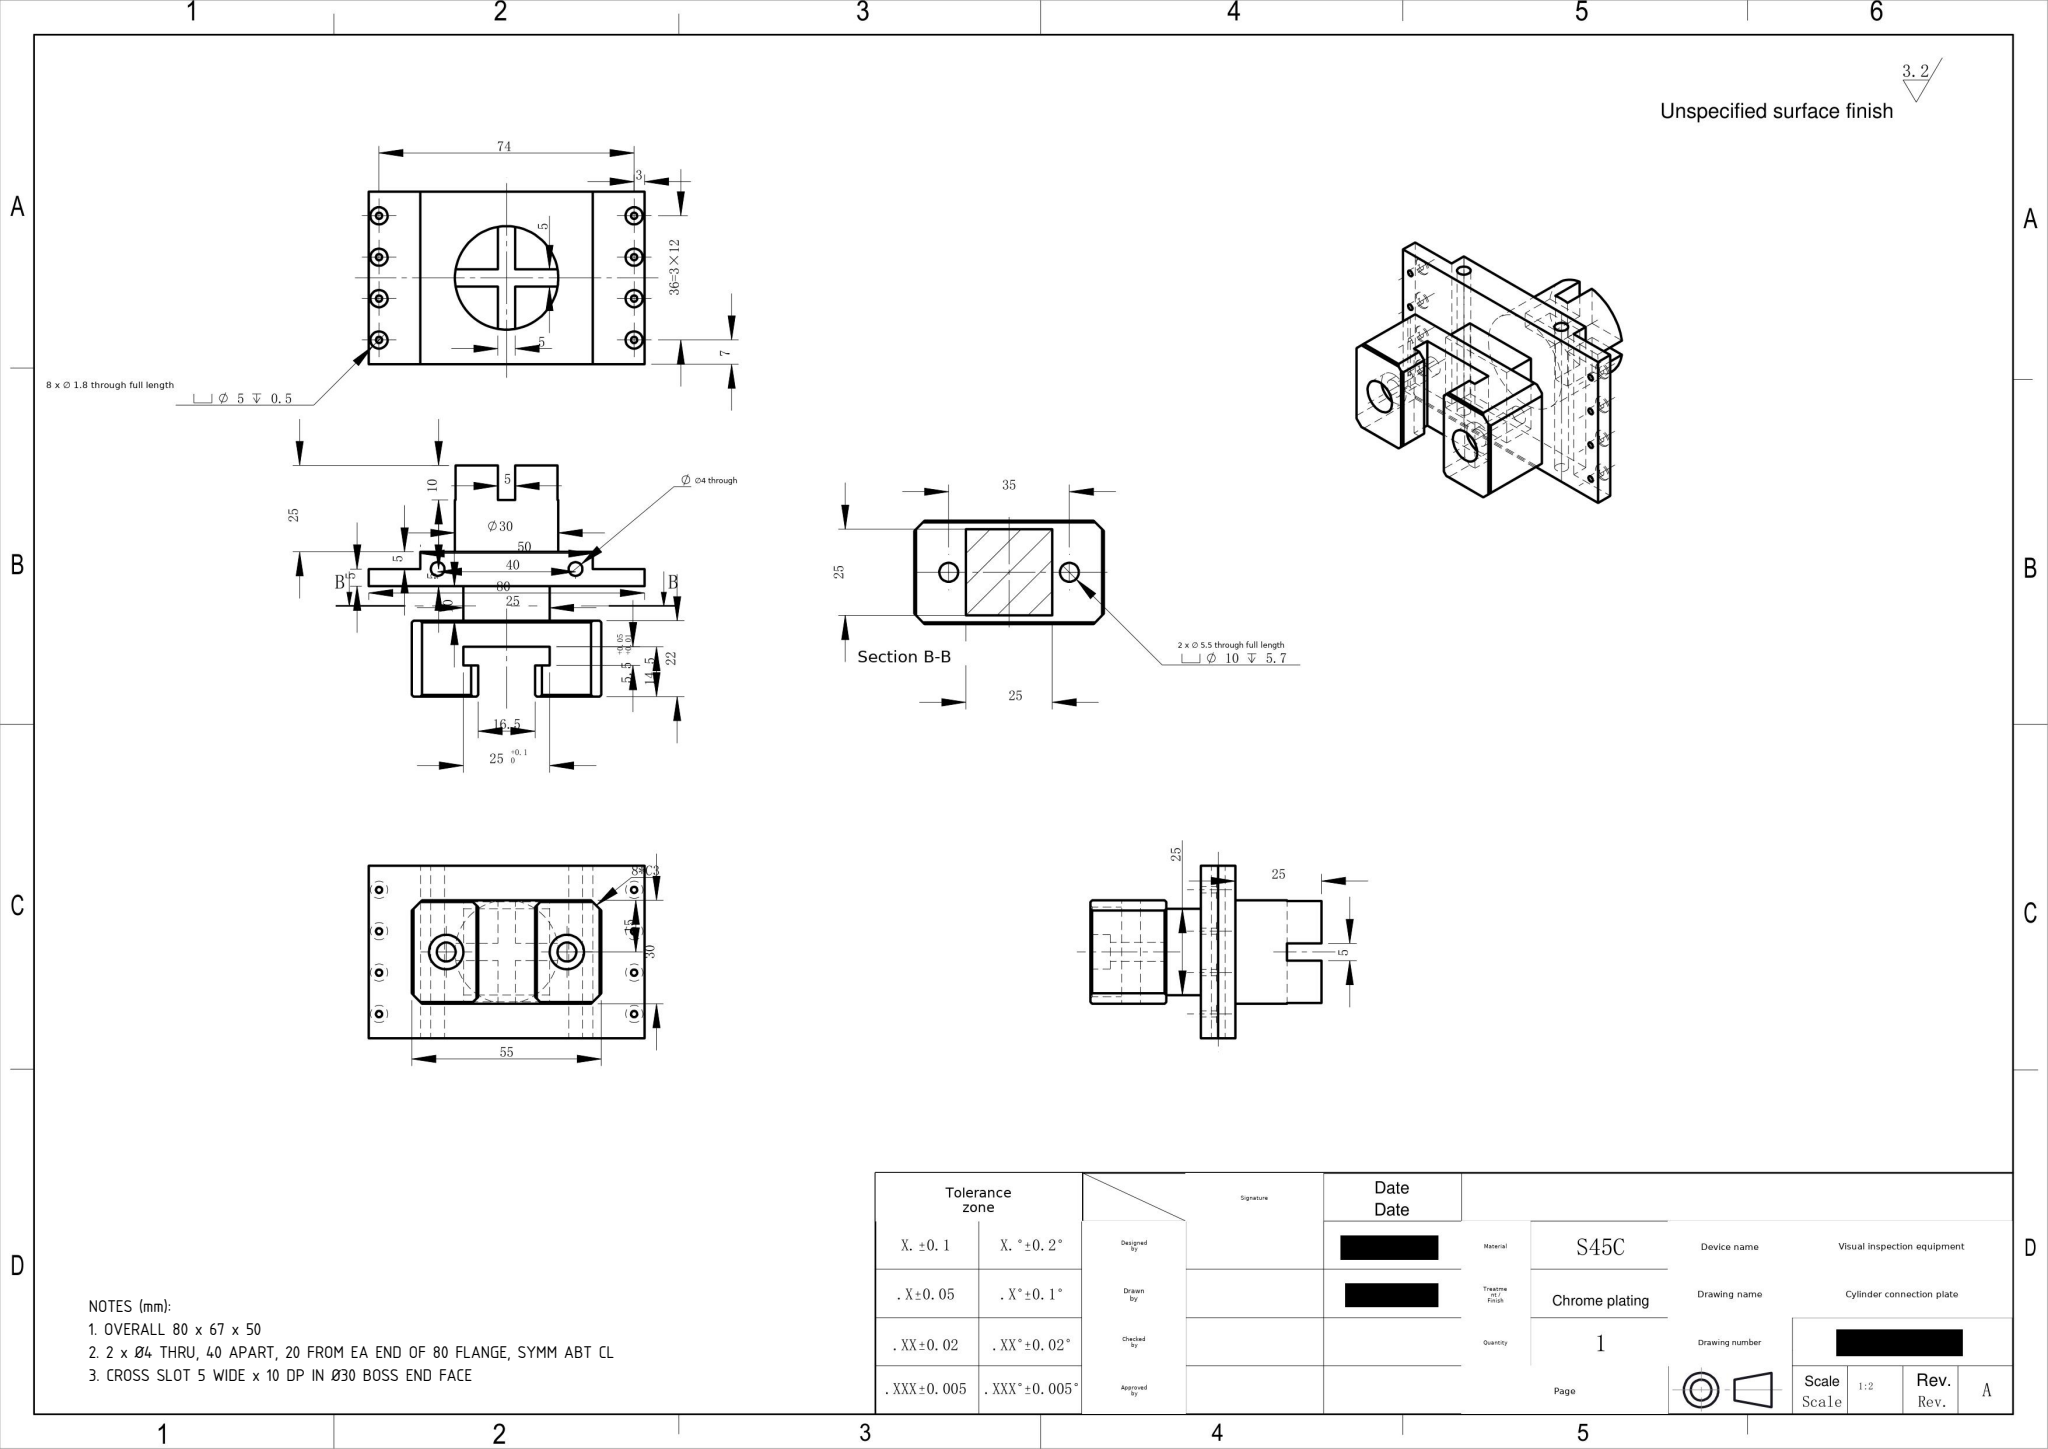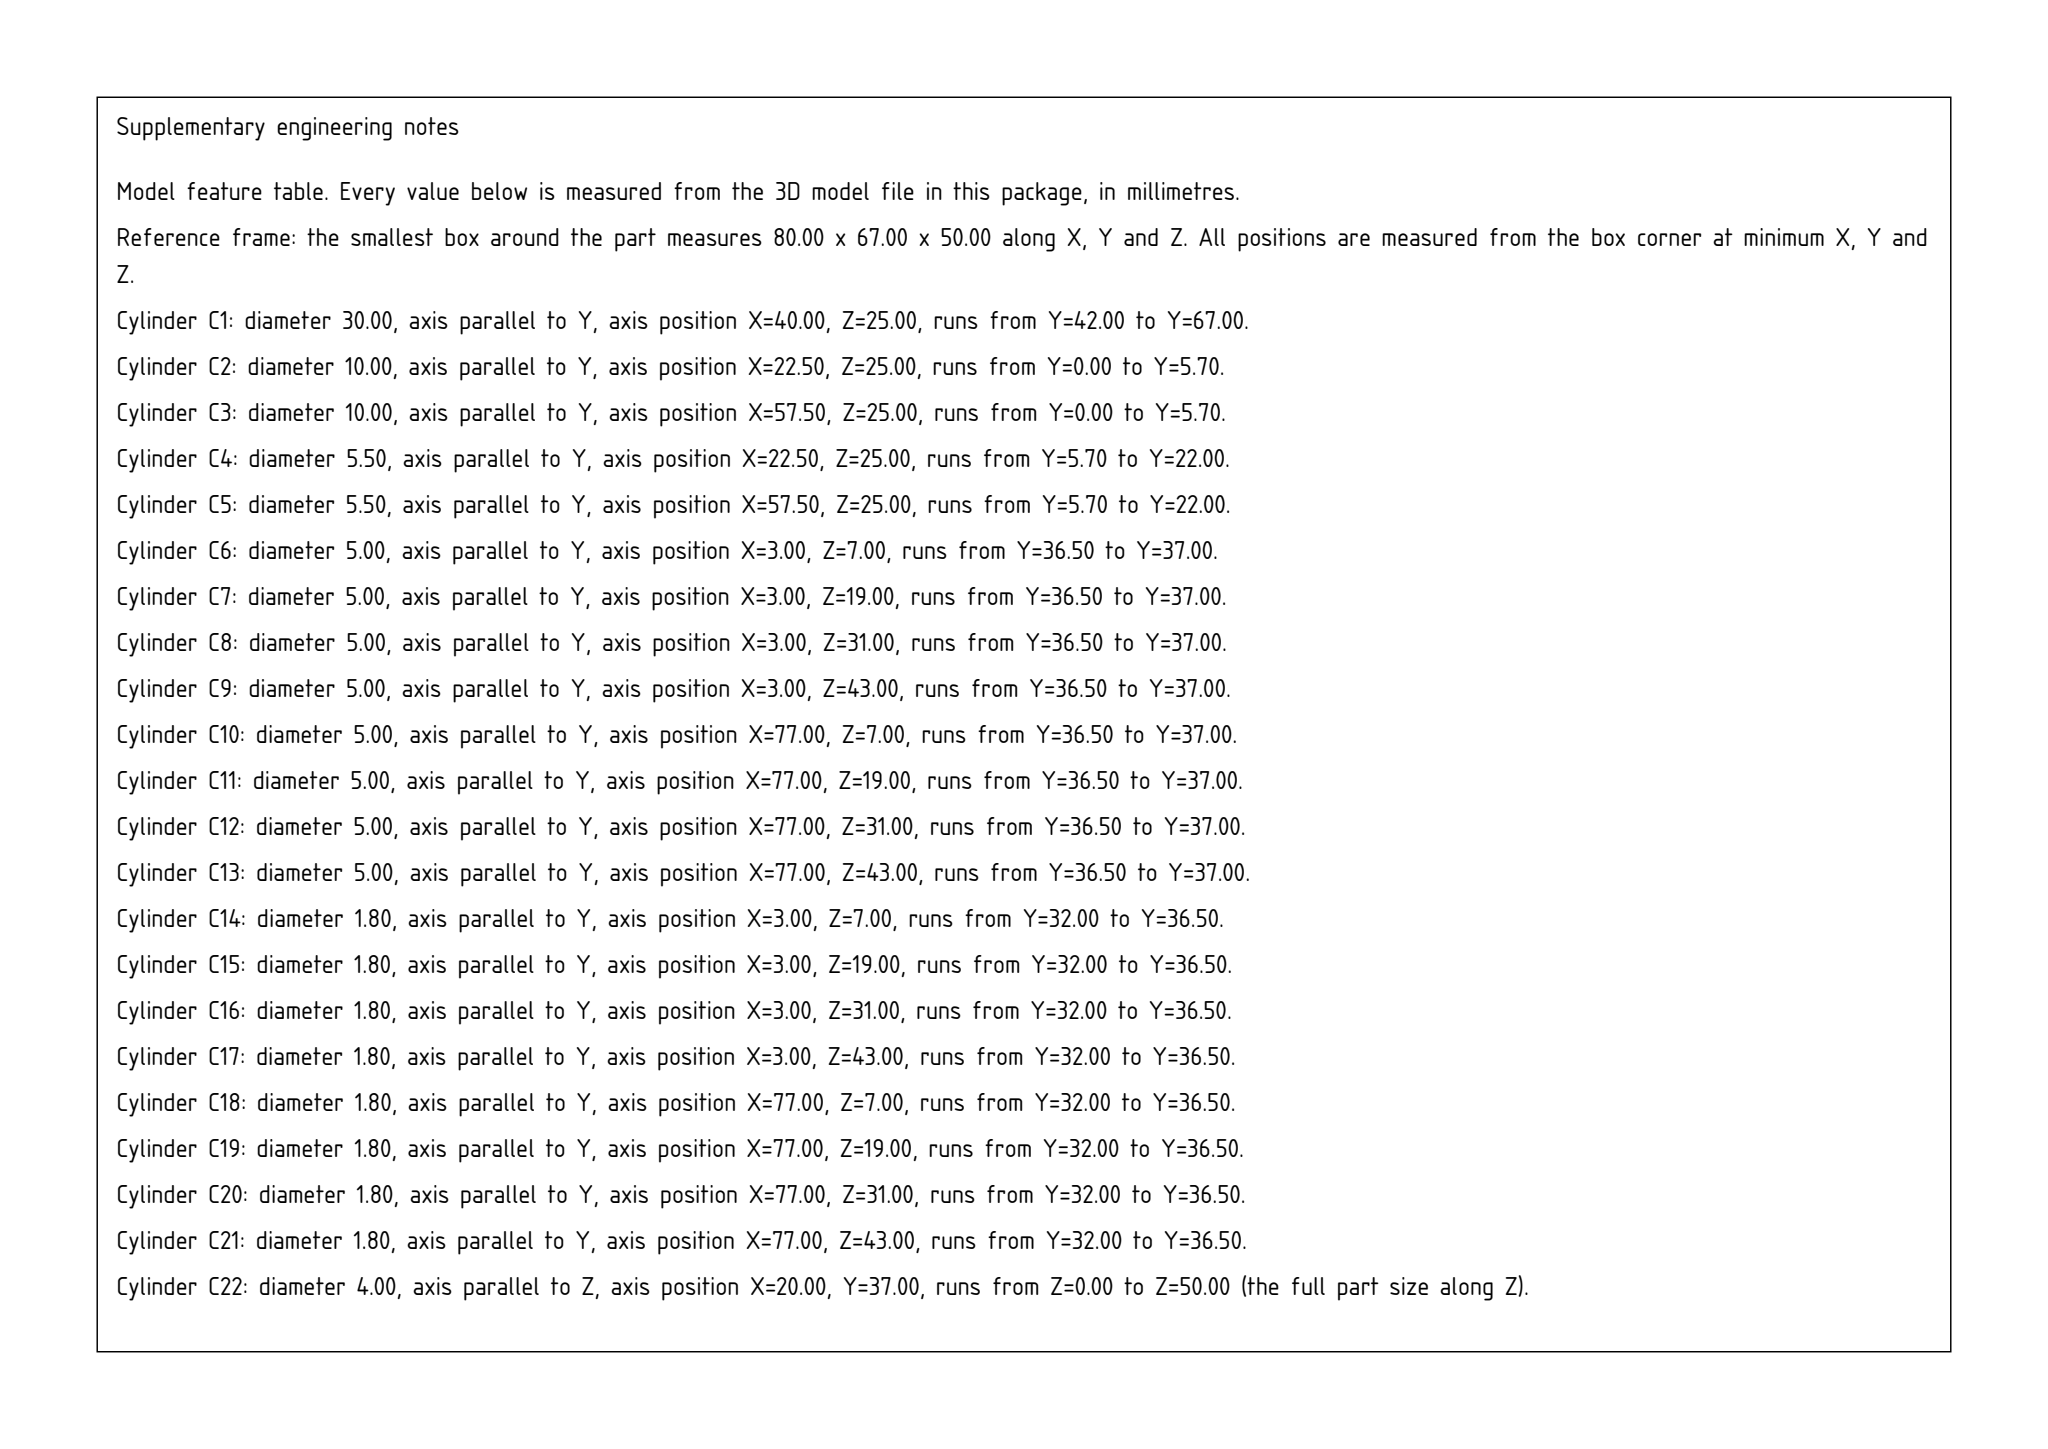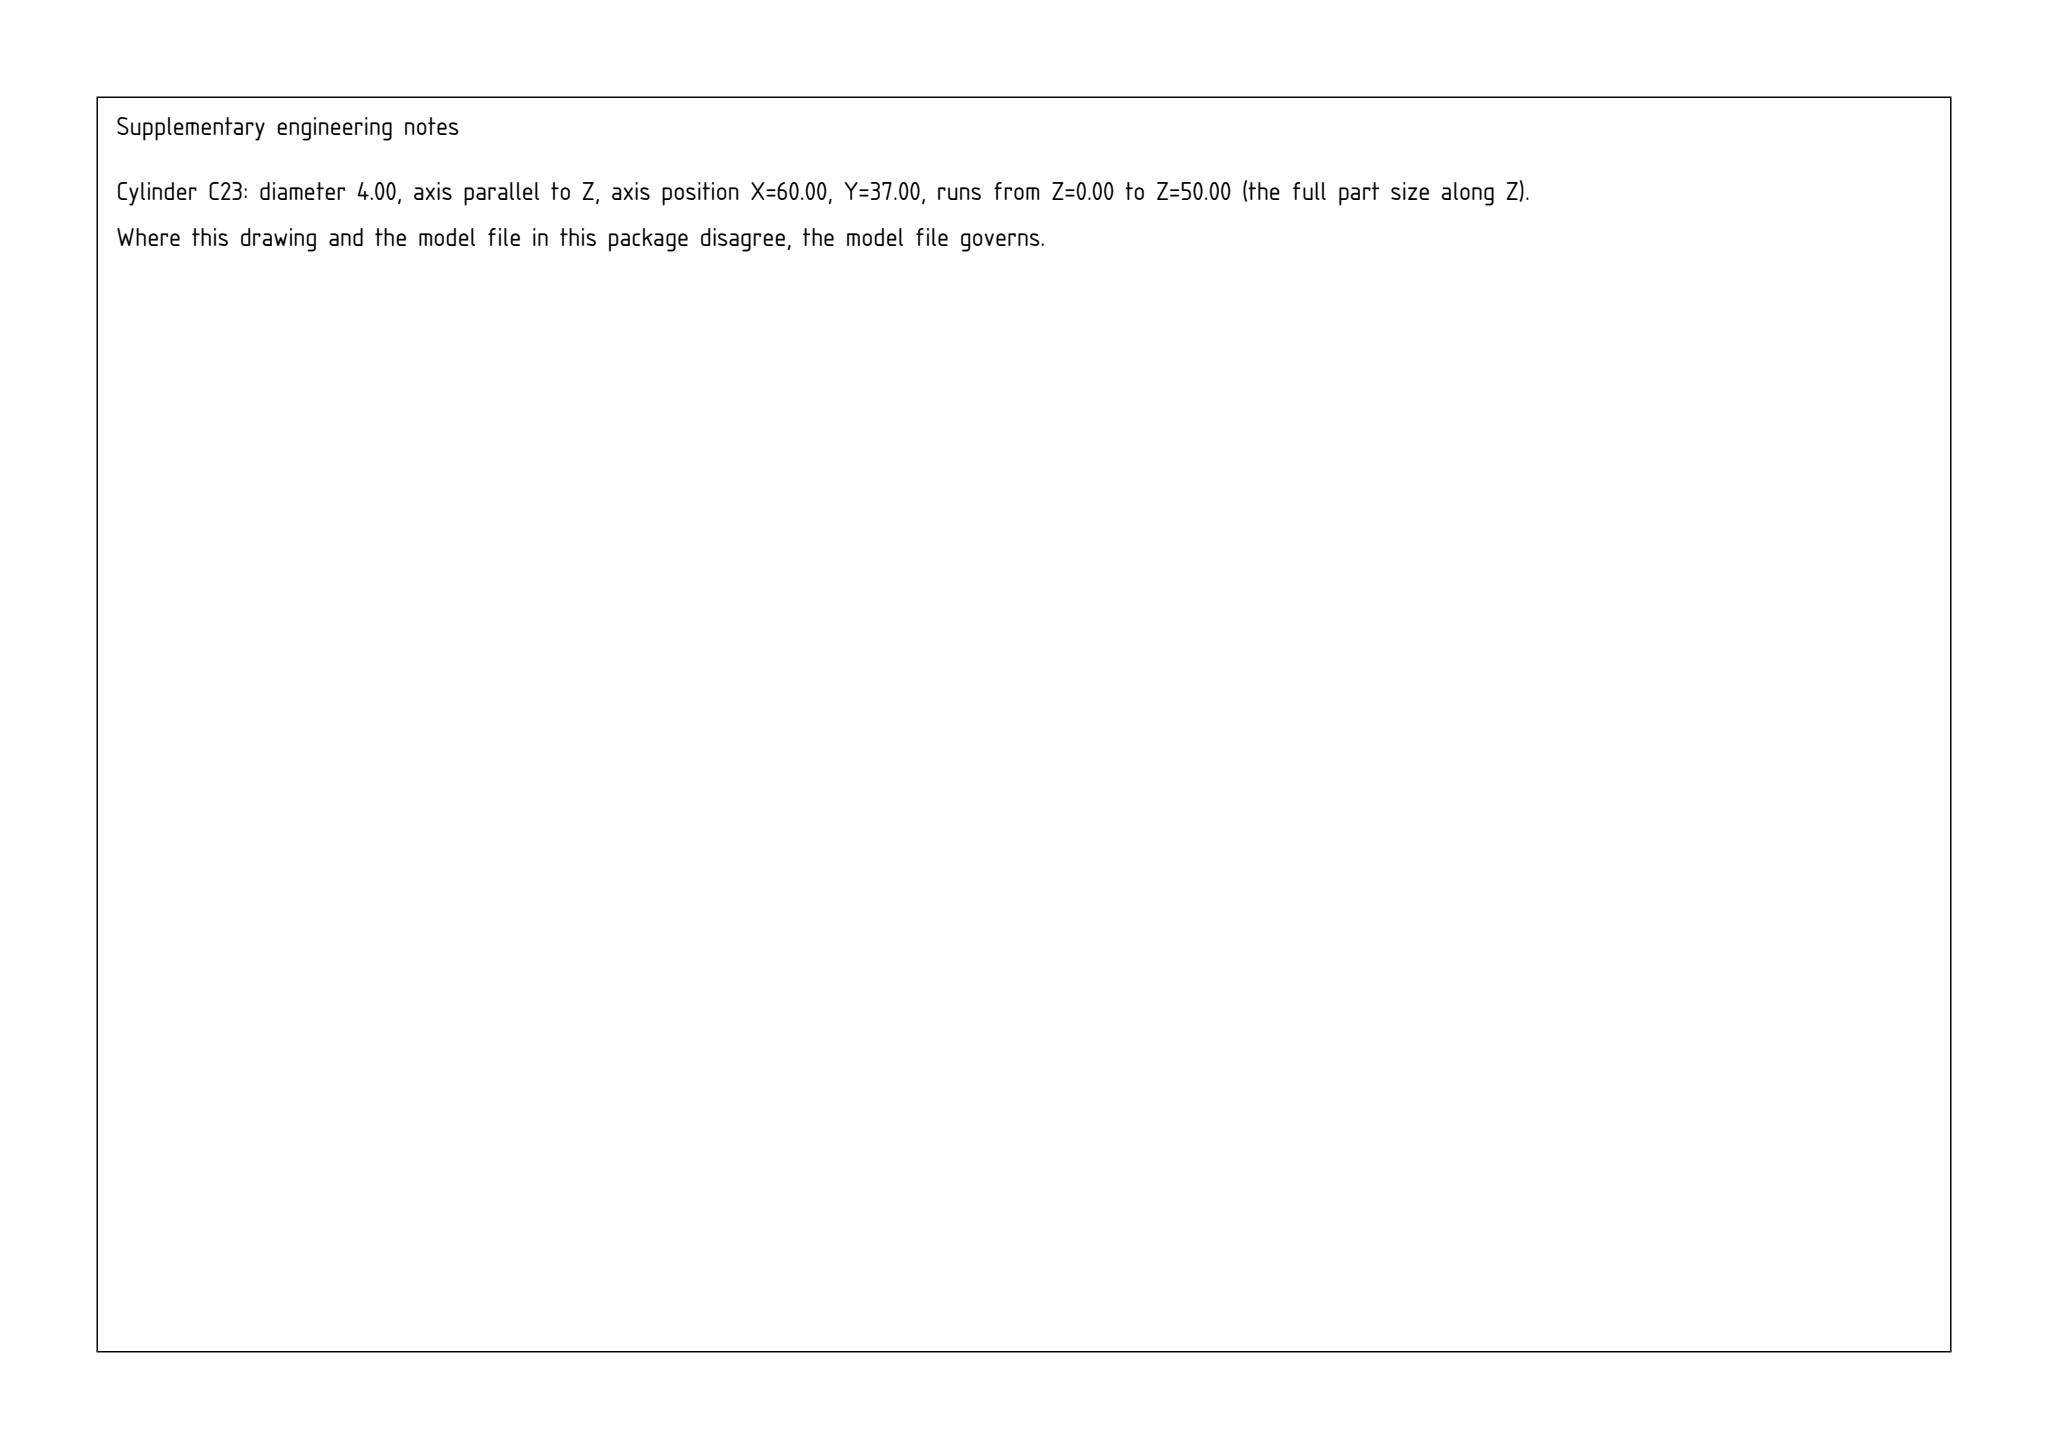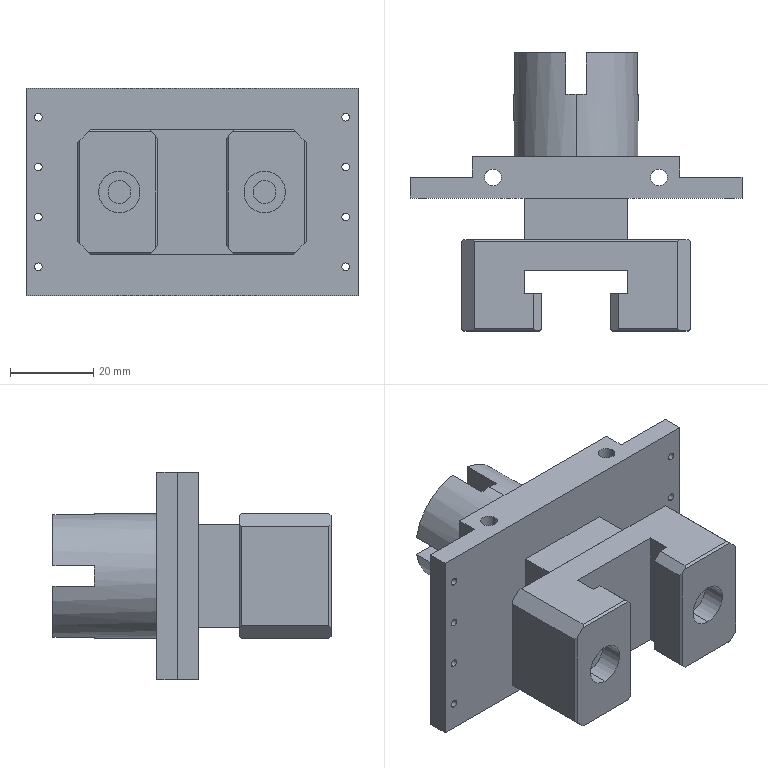Part | SolidWorks | mm | 1 solid | 117 faces | box 80 x 67 x 50 mm | volume 77802 mm3 | plane 71 | cylinder 46 | commonest cylinder face diameters 5 x16 1.8 x16 4 x4 10 x4 5.5 x4 30 x2
Drawing notes:
OVERALL 80 x 67 x 50 | from the solid: bbox_xyz [80.0, 67.0, 50.0]
2 x Ø4 THRU, 40 APART, 20 FROM EA END OF 80 FLANGE, SYMM ABT CL | from the solid: Ø4 cylinders axis z at x=20 & x=60, y=37, length 50 (bbox x=80, CL=40)
CROSS SLOT 5 WIDE x 10 DP IN Ø30 BOSS END FACE | from the solid: Ø30 boss axis y at x=40,z=25 ends at y=67; slot floor plane y=57 -> 10 DP; width 5
build123d program:
from build123d import *

# Parameters (mm, degrees)
BOSS_EXTRUDE1_DEPTH                                  = 15
HOLE_SIZE_ACCORDING_TO_TYPE_1_OF_HEX_S_D             = 5.5
HOLE_SIZE_ACCORDING_TO_TYPE_1_OF_HEX_S_CBORE_D       = 10
HOLE_SIZE_ACCORDING_TO_TYPE_1_OF_HEX_S_CBORE_DEPTH   = 5.7
CHAMFER1_SIZE                                        = 3
CHAMFER2_SIZE                                        = 2
CHAMFER3_SIZE                                        = 0.5
SKETCH4_W                                            = 25
SKETCH4_H                                            = 25
BOSS_EXTRUDE2_DEPTH                                  = 10
SKETCH5_W                                            = 80
SKETCH5_H                                            = 50
BOSS_EXTRUDE3_DEPTH                                  = 10
SKETCH6_R                                            = 15
BOSS_EXTRUDE4_DEPTH                                  = 25
CUT_EXTRUDE1_DEPTH                                   = 10
SKETCH8_W                                            = 15
SKETCH8_H                                            = 5
CUT_EXTRUDE2_DEPTH                                   = 93.677
CYLINDRICAL_COUNTERSUNK_HOLE_FOR_M1_6_HE_D           = 1.8
CYLINDRICAL_COUNTERSUNK_HOLE_FOR_M1_6_HE_CBORE_D     = 5
CYLINDRICAL_COUNTERSUNK_HOLE_FOR_M1_6_HE_CBORE_DEPTH = 0.5
SKETCH12_R                                           = 2
CUT_EXTRUDE3_DEPTH                                   = 93.677


with BuildPart() as part:
    # Sketch1 → Boss-Extrude1 (new, symmetric)
    with BuildSketch(Plane.XY):
        Polygon((-8.25, 0), (-8.25, 9), (-12.5, 9), (-12.5, 14.5), (12.5, 14.5), (12.5, 9), (8.25, 9), (8.25, 0), (27.5, 0), (27.5, 22), (-27.5, 22), (-27.5, 0), align=None)
    extrude(amount=BOSS_EXTRUDE1_DEPTH, both=True)

    # Hole Size _According to_ Type 1 of Hex S (through all)
    with Locations(Plane(origin=(0, 0, 0), x_dir=(-1, 0, 0), z_dir=(0, -1, 0))):
        with Locations((-17.5, 0), (17.5, 0)):
            CounterBoreHole(HOLE_SIZE_ACCORDING_TO_TYPE_1_OF_HEX_S_D / 2, HOLE_SIZE_ACCORDING_TO_TYPE_1_OF_HEX_S_CBORE_D / 2, HOLE_SIZE_ACCORDING_TO_TYPE_1_OF_HEX_S_CBORE_DEPTH)

    # Chamfer1
    chamfer1_edges = [part.edges().sort_by_distance(p)[0] for p in [
        (-27.5, 11, -15),
        (27.5, 11, -15),
        (27.5, 11, 15),
        (-27.5, 11, 15),
    ]]
    chamfer(chamfer1_edges, length=CHAMFER1_SIZE)

    # Chamfer2
    chamfer2_edges = [part.edges().sort_by_distance(p)[0] for p in [
        (8.25, 4.5, -15),
        (-8.25, 4.5, -15),
        (8.25, 4.5, 15),
        (-8.25, 4.5, 15),
    ]]
    chamfer(chamfer2_edges, length=CHAMFER2_SIZE)

    # Chamfer3
    chamfer3_edges = [part.edges().sort_by_distance(p)[0] for p in [
        (27.5, 22, 0),
        (27.5, 0, 0),
        (0, 22, -15),
        (-27.5, 22, 0),
        (0, 22, 15),
        (-17.375, 0, -15),
        (-27.5, 0, 0),
        (-17.375, 0, 15),
        (17.375, 0, 15),
        (-8.25, 0, 0),
        (17.375, 0, -15),
        (8.25, 0, 0),
    ]]
    chamfer(chamfer3_edges, length=CHAMFER3_SIZE)

    # Sketch4 → Boss-Extrude2 (add)
    with BuildSketch(Plane(origin=(0, 22, 0), x_dir=(1, 0, 0), z_dir=(0, 1, 0))):
        Rectangle(SKETCH4_W, SKETCH4_H)
    extrude(amount=BOSS_EXTRUDE2_DEPTH)

    # Sketch5 → Boss-Extrude3 (add)
    with BuildSketch(Plane(origin=(0, 32, 0), x_dir=(1, 0, 0), z_dir=(0, 1, 0))):
        Rectangle(SKETCH5_W, SKETCH5_H)
    extrude(amount=BOSS_EXTRUDE3_DEPTH)

    # Sketch6 → Boss-Extrude4 (add)
    with BuildSketch(Plane(origin=(0, 42, 0), x_dir=(1, 0, 0), z_dir=(0, 1, 0))):
        with Locations(Location((0, 0, 0), (0, 0, 270))):
            Circle(SKETCH6_R)
    extrude(amount=BOSS_EXTRUDE4_DEPTH)

    # Sketch7 → Cut-Extrude1 (cut)
    with BuildSketch(Plane(origin=(0, 67, 0), x_dir=(1, 0, 0), z_dir=(0, 1, 0))):
        Polygon((2.5, 2.5), (20.346, 2.5), (20.346, -2.5), (2.5, -2.5), (2.5, -20.465), (-2.5, -20.465), (-2.5, -2.5), (-20.346, -2.5), (-20.346, 2.5), (-2.5, 2.5), (-2.5, 20.465), (2.5, 20.465), align=None)
    extrude(amount=-CUT_EXTRUDE1_DEPTH, mode=Mode.SUBTRACT)

    # Sketch8 → Cut-Extrude2 (cut, through all)
    with BuildSketch(Plane.XY.offset(25)):
        with Locations((-32.5, 39.5)):
            Rectangle(SKETCH8_W, SKETCH8_H)
        with Locations((32.5, 39.5)):
            Rectangle(SKETCH8_W, SKETCH8_H)
    extrude(amount=-CUT_EXTRUDE2_DEPTH, mode=Mode.SUBTRACT)

    # Cylindrical Countersunk Hole for M1.6 He (through all)
    with Locations(Plane(origin=(0, 37, 0), x_dir=(1, 0, 0), z_dir=(0, 1, 0))):
        with Locations((-37, 18), (-37, 6), (-37, -6), (-37, -18), (37, -18), (37, -6), (37, 6), (37, 18)):
            CounterBoreHole(CYLINDRICAL_COUNTERSUNK_HOLE_FOR_M1_6_HE_D / 2, CYLINDRICAL_COUNTERSUNK_HOLE_FOR_M1_6_HE_CBORE_D / 2, CYLINDRICAL_COUNTERSUNK_HOLE_FOR_M1_6_HE_CBORE_DEPTH)

    # Sketch12 → Cut-Extrude3 (cut, through all)
    with BuildSketch(Plane.XY.offset(25)):
        with Locations((-20, 37)):
            Circle(SKETCH12_R)
        with Locations(Location((20, 37, 0), (0, 0, 180))):
            Circle(SKETCH12_R)
    extrude(amount=-CUT_EXTRUDE3_DEPTH, mode=Mode.SUBTRACT)


solid = part.part